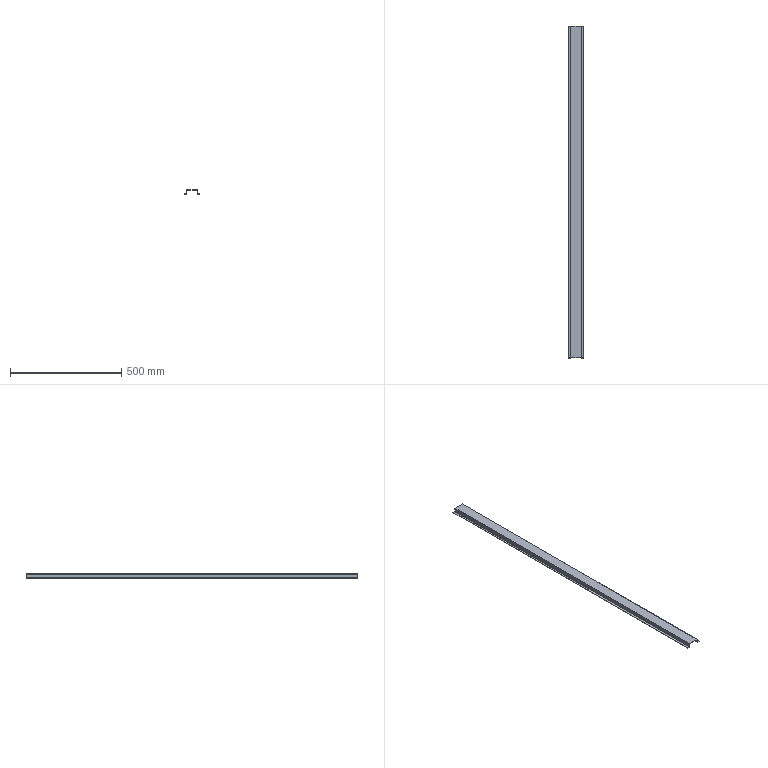Component | SolidWorks | AirFurnaceElectricalCabinet-RearSealingPlateAssembly-1_DoorPanelReinforcementPlate-L1490-1 | 1 solid | 38 faces | box 71.6 x 1490 x 18 mm | volume 183954 mm3 | plane 30 | cylinder 8 | commonest cylinder face diameters 3.9 x4 1.5 x4
STEP:
#1=COLOUR_RGB('',0.7922,0.8196,0.9333);
#2=FILL_AREA_STYLE_COLOUR('',#1);
#3=FILL_AREA_STYLE('',(#2));
#4=SURFACE_STYLE_FILL_AREA(#3);
#5=SURFACE_SIDE_STYLE('',(#4));
#6=SURFACE_STYLE_USAGE(.BOTH.,#5);
#7=PRESENTATION_STYLE_ASSIGNMENT((#6));
#8=CARTESIAN_POINT('',(0.9075,62.795,-9.272));
#9=VERTEX_POINT('',#8);
#10=CARTESIAN_POINT('',(-0.9075,62.795,-9.272));
#11=VERTEX_POINT('',#10);
#12=CARTESIAN_POINT('',(0.9843,62.795,-9.272));
#13=DIRECTION('',(-1.,0.,0.));
#14=VECTOR('',#13,39.37);
#15=LINE('',#12,#14);
#16=EDGE_CURVE('',#9,#11,#15,.T.);
#17=ORIENTED_EDGE('',*,*,#16,.F.);
#18=CARTESIAN_POINT('',(0.9075,62.795,-9.319));
#19=VERTEX_POINT('',#18);
#20=CARTESIAN_POINT('',(0.9075,62.795,-9.272));
#21=DIRECTION('',(0.,-0.,-1.));
#22=VECTOR('',#21,39.37);
#23=LINE('',#20,#22);
#24=EDGE_CURVE('',#9,#19,#23,.T.);
#25=ORIENTED_EDGE('',*,*,#24,.T.);
#26=CARTESIAN_POINT('',(-0.9075,62.795,-9.319));
#27=VERTEX_POINT('',#26);
#28=CARTESIAN_POINT('',(0.9843,62.795,-9.319));
#29=DIRECTION('',(-1.,0.,0.));
#30=VECTOR('',#29,39.37);
#31=LINE('',#28,#30);
#32=EDGE_CURVE('',#19,#27,#31,.T.);
#33=ORIENTED_EDGE('',*,*,#32,.T.);
#34=CARTESIAN_POINT('',(-0.9075,62.795,-9.319));
#35=DIRECTION('',(0.,0.,1.));
#36=VECTOR('',#35,39.37);
#37=LINE('',#34,#36);
#38=EDGE_CURVE('',#27,#11,#37,.T.);
#39=ORIENTED_EDGE('',*,*,#38,.T.);
#40=EDGE_LOOP('',(#17,#25,#33,#39));
#41=FACE_OUTER_BOUND('',#40,.T.);
#42=CARTESIAN_POINT('',(0.937,62.795,-9.348));
#43=DIRECTION('',(0.,1.,-0.));
#44=DIRECTION('',(-1.,0.,0.));
#45=AXIS2_PLACEMENT_3D('',#42,#43,#44);
#46=PLANE('',#45);
#47=ADVANCED_FACE('',(#41),#46,.T.);
#48=CARTESIAN_POINT('',(0.9075,4.134,-9.272));
#49=VERTEX_POINT('',#48);
#50=CARTESIAN_POINT('',(-0.9075,4.134,-9.272));
#51=VERTEX_POINT('',#50);
#52=CARTESIAN_POINT('',(0.9843,4.134,-9.272));
#53=DIRECTION('',(-1.,0.,0.));
#54=VECTOR('',#53,39.37);
#55=LINE('',#52,#54);
#56=EDGE_CURVE('',#49,#51,#55,.T.);
#57=ORIENTED_EDGE('',*,*,#56,.T.);
#58=CARTESIAN_POINT('',(-0.9075,4.134,-9.319));
#59=VERTEX_POINT('',#58);
#60=CARTESIAN_POINT('',(-0.9075,4.134,-9.272));
#61=DIRECTION('',(0.,-0.,-1.));
#62=VECTOR('',#61,39.37);
#63=LINE('',#60,#62);
#64=EDGE_CURVE('',#51,#59,#63,.T.);
#65=ORIENTED_EDGE('',*,*,#64,.T.);
#66=CARTESIAN_POINT('',(0.9075,4.134,-9.319));
#67=VERTEX_POINT('',#66);
#68=CARTESIAN_POINT('',(0.9843,4.134,-9.319));
#69=DIRECTION('',(-1.,0.,0.));
#70=VECTOR('',#69,39.37);
#71=LINE('',#68,#70);
#72=EDGE_CURVE('',#67,#59,#71,.T.);
#73=ORIENTED_EDGE('',*,*,#72,.F.);
#74=CARTESIAN_POINT('',(0.9075,4.134,-9.319));
#75=DIRECTION('',(0.,0.,1.));
#76=VECTOR('',#75,39.37);
#77=LINE('',#74,#76);
#78=EDGE_CURVE('',#67,#49,#77,.T.);
#79=ORIENTED_EDGE('',*,*,#78,.T.);
#80=EDGE_LOOP('',(#57,#65,#73,#79));
#81=FACE_OUTER_BOUND('',#80,.T.);
#82=CARTESIAN_POINT('',(-0.937,4.134,-9.348));
#83=DIRECTION('',(0.,-1.,0.));
#84=DIRECTION('',(1.,0.,0.));
#85=AXIS2_PLACEMENT_3D('',#82,#83,#84);
#86=PLANE('',#85);
#87=ADVANCED_FACE('',(#81),#86,.T.);
#88=ORIENTED_EDGE('',*,*,#56,.F.);
#89=CARTESIAN_POINT('',(0.9075,62.795,-9.272));
#90=DIRECTION('',(0.,-1.,0.));
#91=VECTOR('',#90,39.37);
#92=LINE('',#89,#91);
#93=EDGE_CURVE('',#9,#49,#92,.T.);
#94=ORIENTED_EDGE('',*,*,#93,.F.);
#95=ORIENTED_EDGE('',*,*,#16,.T.);
#96=CARTESIAN_POINT('',(-0.9075,62.795,-9.272));
#97=DIRECTION('',(0.,-1.,0.));
#98=VECTOR('',#97,39.37);
#99=LINE('',#96,#98);
#100=EDGE_CURVE('',#11,#51,#99,.T.);
#101=ORIENTED_EDGE('',*,*,#100,.T.);
#102=EDGE_LOOP('',(#88,#94,#95,#101));
#103=FACE_OUTER_BOUND('',#102,.T.);
#104=CARTESIAN_POINT('',(0.9843,62.795,-9.272));
#105=DIRECTION('',(0.,0.,1.));
#106=DIRECTION('',(1.,0.,0.));
#107=AXIS2_PLACEMENT_3D('',#104,#105,#106);
#108=PLANE('',#107);
#109=ADVANCED_FACE('',(#103),#108,.T.);
#110=ORIENTED_EDGE('',*,*,#72,.T.);
#111=CARTESIAN_POINT('',(-0.9075,62.795,-9.319));
#112=DIRECTION('',(0.,-1.,0.));
#113=VECTOR('',#112,39.37);
#114=LINE('',#111,#113);
#115=EDGE_CURVE('',#27,#59,#114,.T.);
#116=ORIENTED_EDGE('',*,*,#115,.F.);
#117=ORIENTED_EDGE('',*,*,#32,.F.);
#118=CARTESIAN_POINT('',(0.9075,62.795,-9.319));
#119=DIRECTION('',(0.,-1.,0.));
#120=VECTOR('',#119,39.37);
#121=LINE('',#118,#120);
#122=EDGE_CURVE('',#19,#67,#121,.T.);
#123=ORIENTED_EDGE('',*,*,#122,.T.);
#124=EDGE_LOOP('',(#110,#116,#117,#123));
#125=FACE_OUTER_BOUND('',#124,.T.);
#126=CARTESIAN_POINT('',(0.9843,62.795,-9.319));
#127=DIRECTION('',(0.,0.,1.));
#128=DIRECTION('',(1.,0.,0.));
#129=AXIS2_PLACEMENT_3D('',#126,#127,#128);
#130=PLANE('',#129);
#131=ADVANCED_FACE('',(#125),#130,.F.);
#132=ORIENTED_EDGE('',*,*,#38,.F.);
#133=CARTESIAN_POINT('',(-0.937,62.795,-9.348));
#134=VERTEX_POINT('',#133);
#135=CARTESIAN_POINT('',(-0.9075,62.795,-9.348));
#136=DIRECTION('',(0.,-1.,0.));
#137=DIRECTION('',(1.,0.,0.));
#138=AXIS2_PLACEMENT_3D('',#135,#136,#137);
#139=CIRCLE('',#138,0.02953);
#140=EDGE_CURVE('',#27,#134,#139,.T.);
#141=ORIENTED_EDGE('',*,*,#140,.T.);
#142=CARTESIAN_POINT('',(-0.9843,62.795,-9.348));
#143=VERTEX_POINT('',#142);
#144=CARTESIAN_POINT('',(-0.9843,62.795,-9.348));
#145=DIRECTION('',(1.,0.,0.));
#146=VECTOR('',#145,39.37);
#147=LINE('',#144,#146);
#148=EDGE_CURVE('',#143,#134,#147,.T.);
#149=ORIENTED_EDGE('',*,*,#148,.F.);
#150=CARTESIAN_POINT('',(-0.9075,62.795,-9.348));
#151=DIRECTION('',(0.,-1.,0.));
#152=DIRECTION('',(1.,0.,0.));
#153=AXIS2_PLACEMENT_3D('',#150,#151,#152);
#154=CIRCLE('',#153,0.07677);
#155=EDGE_CURVE('',#11,#143,#154,.T.);
#156=ORIENTED_EDGE('',*,*,#155,.F.);
#157=EDGE_LOOP('',(#132,#141,#149,#156));
#158=FACE_OUTER_BOUND('',#157,.T.);
#159=CARTESIAN_POINT('',(-0.9075,62.795,-9.348));
#160=DIRECTION('',(0.,1.,-0.));
#161=DIRECTION('',(-1.,0.,0.));
#162=AXIS2_PLACEMENT_3D('',#159,#160,#161);
#163=PLANE('',#162);
#164=ADVANCED_FACE('',(#158),#163,.T.);
#165=CARTESIAN_POINT('',(-0.937,4.134,-9.348));
#166=VERTEX_POINT('',#165);
#167=CARTESIAN_POINT('',(-0.9843,4.134,-9.348));
#168=VERTEX_POINT('',#167);
#169=CARTESIAN_POINT('',(-0.937,4.134,-9.348));
#170=DIRECTION('',(-1.,0.,0.));
#171=VECTOR('',#170,39.37);
#172=LINE('',#169,#171);
#173=EDGE_CURVE('',#166,#168,#172,.T.);
#174=ORIENTED_EDGE('',*,*,#173,.F.);
#175=CARTESIAN_POINT('',(-0.9075,4.134,-9.348));
#176=DIRECTION('',(0.,1.,-0.));
#177=DIRECTION('',(1.,0.,0.));
#178=AXIS2_PLACEMENT_3D('',#175,#176,#177);
#179=CIRCLE('',#178,0.02953);
#180=EDGE_CURVE('',#166,#59,#179,.T.);
#181=ORIENTED_EDGE('',*,*,#180,.T.);
#182=ORIENTED_EDGE('',*,*,#64,.F.);
#183=CARTESIAN_POINT('',(-0.9075,4.134,-9.348));
#184=DIRECTION('',(0.,1.,-0.));
#185=DIRECTION('',(-1.,0.,0.));
#186=AXIS2_PLACEMENT_3D('',#183,#184,#185);
#187=CIRCLE('',#186,0.07677);
#188=EDGE_CURVE('',#168,#51,#187,.T.);
#189=ORIENTED_EDGE('',*,*,#188,.F.);
#190=EDGE_LOOP('',(#174,#181,#182,#189));
#191=FACE_OUTER_BOUND('',#190,.T.);
#192=CARTESIAN_POINT('',(-0.9075,4.134,-9.348));
#193=DIRECTION('',(0.,-1.,0.));
#194=DIRECTION('',(1.,0.,0.));
#195=AXIS2_PLACEMENT_3D('',#192,#193,#194);
#196=PLANE('',#195);
#197=ADVANCED_FACE('',(#191),#196,.T.);
#198=ORIENTED_EDGE('',*,*,#188,.T.);
#199=ORIENTED_EDGE('',*,*,#100,.F.);
#200=ORIENTED_EDGE('',*,*,#155,.T.);
#201=CARTESIAN_POINT('',(-0.9843,62.795,-9.348));
#202=DIRECTION('',(0.,-1.,0.));
#203=VECTOR('',#202,39.37);
#204=LINE('',#201,#203);
#205=EDGE_CURVE('',#143,#168,#204,.T.);
#206=ORIENTED_EDGE('',*,*,#205,.T.);
#207=EDGE_LOOP('',(#198,#199,#200,#206));
#208=FACE_OUTER_BOUND('',#207,.T.);
#209=CARTESIAN_POINT('',(-0.9075,92.126,-9.348));
#210=DIRECTION('',(0.,-1.,0.));
#211=DIRECTION('',(1.,0.,0.));
#212=AXIS2_PLACEMENT_3D('',#209,#210,#211);
#213=CYLINDRICAL_SURFACE('',#212,0.07677);
#214=ADVANCED_FACE('',(#208),#213,.T.);
#215=ORIENTED_EDGE('',*,*,#180,.F.);
#216=CARTESIAN_POINT('',(-0.937,62.795,-9.348));
#217=DIRECTION('',(0.,-1.,0.));
#218=VECTOR('',#217,39.37);
#219=LINE('',#216,#218);
#220=EDGE_CURVE('',#134,#166,#219,.T.);
#221=ORIENTED_EDGE('',*,*,#220,.F.);
#222=ORIENTED_EDGE('',*,*,#140,.F.);
#223=ORIENTED_EDGE('',*,*,#115,.T.);
#224=EDGE_LOOP('',(#215,#221,#222,#223));
#225=FACE_OUTER_BOUND('',#224,.T.);
#226=CARTESIAN_POINT('',(-0.9075,92.126,-9.348));
#227=DIRECTION('',(0.,-1.,0.));
#228=DIRECTION('',(1.,0.,0.));
#229=AXIS2_PLACEMENT_3D('',#226,#227,#228);
#230=CYLINDRICAL_SURFACE('',#229,0.02953);
#231=ADVANCED_FACE('',(#225),#230,.F.);
#232=CARTESIAN_POINT('',(-1.409,4.134,-9.933));
#233=VERTEX_POINT('',#232);
#234=CARTESIAN_POINT('',(-1.409,4.134,-9.98));
#235=VERTEX_POINT('',#234);
#236=CARTESIAN_POINT('',(-1.409,4.134,-9.933));
#237=DIRECTION('',(0.,-0.,-1.));
#238=VECTOR('',#237,39.37);
#239=LINE('',#236,#238);
#240=EDGE_CURVE('',#233,#235,#239,.T.);
#241=ORIENTED_EDGE('',*,*,#240,.F.);
#242=CARTESIAN_POINT('',(-1.409,62.795,-9.933));
#243=VERTEX_POINT('',#242);
#244=CARTESIAN_POINT('',(-1.409,62.795,-9.933));
#245=DIRECTION('',(0.,-1.,0.));
#246=VECTOR('',#245,39.37);
#247=LINE('',#244,#246);
#248=EDGE_CURVE('',#243,#233,#247,.T.);
#249=ORIENTED_EDGE('',*,*,#248,.F.);
#250=CARTESIAN_POINT('',(-1.409,62.795,-9.98));
#251=VERTEX_POINT('',#250);
#252=CARTESIAN_POINT('',(-1.409,62.795,-9.933));
#253=DIRECTION('',(0.,-0.,-1.));
#254=VECTOR('',#253,39.37);
#255=LINE('',#252,#254);
#256=EDGE_CURVE('',#243,#251,#255,.T.);
#257=ORIENTED_EDGE('',*,*,#256,.T.);
#258=CARTESIAN_POINT('',(-1.409,62.795,-9.98));
#259=DIRECTION('',(0.,-1.,0.));
#260=VECTOR('',#259,39.37);
#261=LINE('',#258,#260);
#262=EDGE_CURVE('',#251,#235,#261,.T.);
#263=ORIENTED_EDGE('',*,*,#262,.T.);
#264=EDGE_LOOP('',(#241,#249,#257,#263));
#265=FACE_OUTER_BOUND('',#264,.T.);
#266=CARTESIAN_POINT('',(-1.409,62.795,-9.933));
#267=DIRECTION('',(-1.,0.,0.));
#268=DIRECTION('',(0.,-1.,0.));
#269=AXIS2_PLACEMENT_3D('',#266,#267,#268);
#270=PLANE('',#269);
#271=ADVANCED_FACE('',(#265),#270,.T.);
#272=CARTESIAN_POINT('',(-1.014,4.134,-9.98));
#273=VERTEX_POINT('',#272);
#274=CARTESIAN_POINT('',(-0.9843,4.134,-9.98));
#275=DIRECTION('',(-1.,0.,0.));
#276=VECTOR('',#275,39.37);
#277=LINE('',#274,#276);
#278=EDGE_CURVE('',#273,#235,#277,.T.);
#279=ORIENTED_EDGE('',*,*,#278,.F.);
#280=CARTESIAN_POINT('',(-1.014,4.134,-9.933));
#281=VERTEX_POINT('',#280);
#282=CARTESIAN_POINT('',(-1.014,4.134,-9.98));
#283=DIRECTION('',(0.,0.,1.));
#284=VECTOR('',#283,39.37);
#285=LINE('',#282,#284);
#286=EDGE_CURVE('',#273,#281,#285,.T.);
#287=ORIENTED_EDGE('',*,*,#286,.T.);
#288=CARTESIAN_POINT('',(-0.9843,4.134,-9.933));
#289=DIRECTION('',(-1.,0.,0.));
#290=VECTOR('',#289,39.37);
#291=LINE('',#288,#290);
#292=EDGE_CURVE('',#281,#233,#291,.T.);
#293=ORIENTED_EDGE('',*,*,#292,.T.);
#294=ORIENTED_EDGE('',*,*,#240,.T.);
#295=EDGE_LOOP('',(#279,#287,#293,#294));
#296=FACE_OUTER_BOUND('',#295,.T.);
#297=CARTESIAN_POINT('',(-1.014,4.134,-9.904));
#298=DIRECTION('',(0.,-1.,0.));
#299=DIRECTION('',(1.,0.,0.));
#300=AXIS2_PLACEMENT_3D('',#297,#298,#299);
#301=PLANE('',#300);
#302=ADVANCED_FACE('',(#296),#301,.T.);
#303=ORIENTED_EDGE('',*,*,#278,.T.);
#304=ORIENTED_EDGE('',*,*,#262,.F.);
#305=CARTESIAN_POINT('',(-1.014,62.795,-9.98));
#306=VERTEX_POINT('',#305);
#307=CARTESIAN_POINT('',(-0.9843,62.795,-9.98));
#308=DIRECTION('',(-1.,0.,0.));
#309=VECTOR('',#308,39.37);
#310=LINE('',#307,#309);
#311=EDGE_CURVE('',#306,#251,#310,.T.);
#312=ORIENTED_EDGE('',*,*,#311,.F.);
#313=CARTESIAN_POINT('',(-1.014,62.795,-9.98));
#314=DIRECTION('',(0.,-1.,0.));
#315=VECTOR('',#314,39.37);
#316=LINE('',#313,#315);
#317=EDGE_CURVE('',#306,#273,#316,.T.);
#318=ORIENTED_EDGE('',*,*,#317,.T.);
#319=EDGE_LOOP('',(#303,#304,#312,#318));
#320=FACE_OUTER_BOUND('',#319,.T.);
#321=CARTESIAN_POINT('',(-0.9843,62.795,-9.98));
#322=DIRECTION('',(0.,0.,1.));
#323=DIRECTION('',(1.,-0.,-0.));
#324=AXIS2_PLACEMENT_3D('',#321,#322,#323);
#325=PLANE('',#324);
#326=ADVANCED_FACE('',(#320),#325,.F.);
#327=CARTESIAN_POINT('',(-1.014,62.795,-9.933));
#328=VERTEX_POINT('',#327);
#329=CARTESIAN_POINT('',(-0.9843,62.795,-9.933));
#330=DIRECTION('',(-1.,0.,0.));
#331=VECTOR('',#330,39.37);
#332=LINE('',#329,#331);
#333=EDGE_CURVE('',#328,#243,#332,.T.);
#334=ORIENTED_EDGE('',*,*,#333,.F.);
#335=CARTESIAN_POINT('',(-1.014,62.795,-9.933));
#336=DIRECTION('',(0.,-0.,-1.));
#337=VECTOR('',#336,39.37);
#338=LINE('',#335,#337);
#339=EDGE_CURVE('',#328,#306,#338,.T.);
#340=ORIENTED_EDGE('',*,*,#339,.T.);
#341=ORIENTED_EDGE('',*,*,#311,.T.);
#342=ORIENTED_EDGE('',*,*,#256,.F.);
#343=EDGE_LOOP('',(#334,#340,#341,#342));
#344=FACE_OUTER_BOUND('',#343,.T.);
#345=CARTESIAN_POINT('',(-0.937,62.795,-9.904));
#346=DIRECTION('',(0.,1.,-0.));
#347=DIRECTION('',(-1.,0.,0.));
#348=AXIS2_PLACEMENT_3D('',#345,#346,#347);
#349=PLANE('',#348);
#350=ADVANCED_FACE('',(#344),#349,.T.);
#351=ORIENTED_EDGE('',*,*,#292,.F.);
#352=CARTESIAN_POINT('',(-1.014,62.795,-9.933));
#353=DIRECTION('',(0.,-1.,0.));
#354=VECTOR('',#353,39.37);
#355=LINE('',#352,#354);
#356=EDGE_CURVE('',#328,#281,#355,.T.);
#357=ORIENTED_EDGE('',*,*,#356,.F.);
#358=ORIENTED_EDGE('',*,*,#333,.T.);
#359=ORIENTED_EDGE('',*,*,#248,.T.);
#360=EDGE_LOOP('',(#351,#357,#358,#359));
#361=FACE_OUTER_BOUND('',#360,.T.);
#362=CARTESIAN_POINT('',(-0.9843,62.795,-9.933));
#363=DIRECTION('',(0.,0.,1.));
#364=DIRECTION('',(1.,-0.,-0.));
#365=AXIS2_PLACEMENT_3D('',#362,#363,#364);
#366=PLANE('',#365);
#367=ADVANCED_FACE('',(#361),#366,.T.);
#368=ORIENTED_EDGE('',*,*,#286,.F.);
#369=CARTESIAN_POINT('',(-0.937,4.134,-9.904));
#370=VERTEX_POINT('',#369);
#371=CARTESIAN_POINT('',(-1.014,4.134,-9.904));
#372=DIRECTION('',(0.,-1.,0.));
#373=DIRECTION('',(0.,0.,1.));
#374=AXIS2_PLACEMENT_3D('',#371,#372,#373);
#375=CIRCLE('',#374,0.07677);
#376=EDGE_CURVE('',#273,#370,#375,.T.);
#377=ORIENTED_EDGE('',*,*,#376,.T.);
#378=CARTESIAN_POINT('',(-0.9843,4.134,-9.904));
#379=VERTEX_POINT('',#378);
#380=CARTESIAN_POINT('',(-0.9843,4.134,-9.904));
#381=DIRECTION('',(1.,0.,0.));
#382=VECTOR('',#381,39.37);
#383=LINE('',#380,#382);
#384=EDGE_CURVE('',#379,#370,#383,.T.);
#385=ORIENTED_EDGE('',*,*,#384,.F.);
#386=CARTESIAN_POINT('',(-1.014,4.134,-9.904));
#387=DIRECTION('',(0.,-1.,0.));
#388=DIRECTION('',(0.,0.,1.));
#389=AXIS2_PLACEMENT_3D('',#386,#387,#388);
#390=CIRCLE('',#389,0.02953);
#391=EDGE_CURVE('',#281,#379,#390,.T.);
#392=ORIENTED_EDGE('',*,*,#391,.F.);
#393=EDGE_LOOP('',(#368,#377,#385,#392));
#394=FACE_OUTER_BOUND('',#393,.T.);
#395=CARTESIAN_POINT('',(-1.014,4.134,-9.904));
#396=DIRECTION('',(0.,1.,-0.));
#397=DIRECTION('',(-0.,-0.,-1.));
#398=AXIS2_PLACEMENT_3D('',#395,#396,#397);
#399=PLANE('',#398);
#400=ADVANCED_FACE('',(#394),#399,.F.);
#401=ORIENTED_EDGE('',*,*,#376,.F.);
#402=ORIENTED_EDGE('',*,*,#317,.F.);
#403=CARTESIAN_POINT('',(-0.937,62.795,-9.904));
#404=VERTEX_POINT('',#403);
#405=CARTESIAN_POINT('',(-1.014,62.795,-9.904));
#406=DIRECTION('',(0.,1.,-0.));
#407=DIRECTION('',(0.,0.,1.));
#408=AXIS2_PLACEMENT_3D('',#405,#406,#407);
#409=CIRCLE('',#408,0.07677);
#410=EDGE_CURVE('',#404,#306,#409,.T.);
#411=ORIENTED_EDGE('',*,*,#410,.F.);
#412=CARTESIAN_POINT('',(-0.937,62.795,-9.904));
#413=DIRECTION('',(0.,-1.,0.));
#414=VECTOR('',#413,39.37);
#415=LINE('',#412,#414);
#416=EDGE_CURVE('',#404,#370,#415,.T.);
#417=ORIENTED_EDGE('',*,*,#416,.T.);
#418=EDGE_LOOP('',(#401,#402,#411,#417));
#419=FACE_OUTER_BOUND('',#418,.T.);
#420=CARTESIAN_POINT('',(-1.014,92.126,-9.904));
#421=DIRECTION('',(0.,-1.,0.));
#422=DIRECTION('',(0.,0.,1.));
#423=AXIS2_PLACEMENT_3D('',#420,#421,#422);
#424=CYLINDRICAL_SURFACE('',#423,0.07677);
#425=ADVANCED_FACE('',(#419),#424,.T.);
#426=CARTESIAN_POINT('',(-0.9843,62.795,-9.904));
#427=VERTEX_POINT('',#426);
#428=CARTESIAN_POINT('',(-0.937,62.795,-9.904));
#429=DIRECTION('',(-1.,-0.,-0.));
#430=VECTOR('',#429,39.37);
#431=LINE('',#428,#430);
#432=EDGE_CURVE('',#404,#427,#431,.T.);
#433=ORIENTED_EDGE('',*,*,#432,.F.);
#434=ORIENTED_EDGE('',*,*,#410,.T.);
#435=ORIENTED_EDGE('',*,*,#339,.F.);
#436=CARTESIAN_POINT('',(-1.014,62.795,-9.904));
#437=DIRECTION('',(0.,1.,-0.));
#438=DIRECTION('',(0.,0.,-1.));
#439=AXIS2_PLACEMENT_3D('',#436,#437,#438);
#440=CIRCLE('',#439,0.02953);
#441=EDGE_CURVE('',#427,#328,#440,.T.);
#442=ORIENTED_EDGE('',*,*,#441,.F.);
#443=EDGE_LOOP('',(#433,#434,#435,#442));
#444=FACE_OUTER_BOUND('',#443,.T.);
#445=CARTESIAN_POINT('',(-1.014,62.795,-9.904));
#446=DIRECTION('',(0.,-1.,0.));
#447=DIRECTION('',(0.,0.,1.));
#448=AXIS2_PLACEMENT_3D('',#445,#446,#447);
#449=PLANE('',#448);
#450=ADVANCED_FACE('',(#444),#449,.F.);
#451=ORIENTED_EDGE('',*,*,#391,.T.);
#452=CARTESIAN_POINT('',(-0.9843,62.795,-9.904));
#453=DIRECTION('',(0.,-1.,0.));
#454=VECTOR('',#453,39.37);
#455=LINE('',#452,#454);
#456=EDGE_CURVE('',#427,#379,#455,.T.);
#457=ORIENTED_EDGE('',*,*,#456,.F.);
#458=ORIENTED_EDGE('',*,*,#441,.T.);
#459=ORIENTED_EDGE('',*,*,#356,.T.);
#460=EDGE_LOOP('',(#451,#457,#458,#459));
#461=FACE_OUTER_BOUND('',#460,.T.);
#462=CARTESIAN_POINT('',(-1.014,92.126,-9.904));
#463=DIRECTION('',(0.,-1.,0.));
#464=DIRECTION('',(0.,0.,1.));
#465=AXIS2_PLACEMENT_3D('',#462,#463,#464);
#466=CYLINDRICAL_SURFACE('',#465,0.02953);
#467=ADVANCED_FACE('',(#461),#466,.F.);
#468=CARTESIAN_POINT('',(-0.9843,4.134,-9.272));
#469=DIRECTION('',(0.,-0.,-1.));
#470=VECTOR('',#469,39.37);
#471=LINE('',#468,#470);
#472=EDGE_CURVE('',#168,#379,#471,.T.);
#473=ORIENTED_EDGE('',*,*,#472,.F.);
#474=ORIENTED_EDGE('',*,*,#205,.F.);
#475=CARTESIAN_POINT('',(-0.9843,62.795,-9.272));
#476=DIRECTION('',(0.,-0.,-1.));
#477=VECTOR('',#476,39.37);
#478=LINE('',#475,#477);
#479=EDGE_CURVE('',#143,#427,#478,.T.);
#480=ORIENTED_EDGE('',*,*,#479,.T.);
#481=ORIENTED_EDGE('',*,*,#456,.T.);
#482=EDGE_LOOP('',(#473,#474,#480,#481));
#483=FACE_OUTER_BOUND('',#482,.T.);
#484=CARTESIAN_POINT('',(-0.9843,62.795,-9.272));
#485=DIRECTION('',(-1.,0.,0.));
#486=DIRECTION('',(0.,-1.,0.));
#487=AXIS2_PLACEMENT_3D('',#484,#485,#486);
#488=PLANE('',#487);
#489=ADVANCED_FACE('',(#483),#488,.T.);
#490=ORIENTED_EDGE('',*,*,#479,.F.);
#491=ORIENTED_EDGE('',*,*,#148,.T.);
#492=CARTESIAN_POINT('',(-0.937,62.795,-9.272));
#493=DIRECTION('',(0.,-0.,-1.));
#494=VECTOR('',#493,39.37);
#495=LINE('',#492,#494);
#496=EDGE_CURVE('',#134,#404,#495,.T.);
#497=ORIENTED_EDGE('',*,*,#496,.T.);
#498=ORIENTED_EDGE('',*,*,#432,.T.);
#499=EDGE_LOOP('',(#490,#491,#497,#498));
#500=FACE_OUTER_BOUND('',#499,.T.);
#501=CARTESIAN_POINT('',(-0.9075,62.795,-9.319));
#502=DIRECTION('',(0.,1.,-0.));
#503=DIRECTION('',(-1.,0.,0.));
#504=AXIS2_PLACEMENT_3D('',#501,#502,#503);
#505=PLANE('',#504);
#506=ADVANCED_FACE('',(#500),#505,.T.);
#507=CARTESIAN_POINT('',(-0.937,4.134,-9.272));
#508=DIRECTION('',(0.,-0.,-1.));
#509=VECTOR('',#508,39.37);
#510=LINE('',#507,#509);
#511=EDGE_CURVE('',#166,#370,#510,.T.);
#512=ORIENTED_EDGE('',*,*,#511,.T.);
#513=ORIENTED_EDGE('',*,*,#416,.F.);
#514=ORIENTED_EDGE('',*,*,#496,.F.);
#515=ORIENTED_EDGE('',*,*,#220,.T.);
#516=EDGE_LOOP('',(#512,#513,#514,#515));
#517=FACE_OUTER_BOUND('',#516,.T.);
#518=CARTESIAN_POINT('',(-0.937,62.795,-9.272));
#519=DIRECTION('',(-1.,0.,0.));
#520=DIRECTION('',(0.,-1.,0.));
#521=AXIS2_PLACEMENT_3D('',#518,#519,#520);
#522=PLANE('',#521);
#523=ADVANCED_FACE('',(#517),#522,.F.);
#524=ORIENTED_EDGE('',*,*,#472,.T.);
#525=ORIENTED_EDGE('',*,*,#384,.T.);
#526=ORIENTED_EDGE('',*,*,#511,.F.);
#527=ORIENTED_EDGE('',*,*,#173,.T.);
#528=EDGE_LOOP('',(#524,#525,#526,#527));
#529=FACE_OUTER_BOUND('',#528,.T.);
#530=CARTESIAN_POINT('',(-1.014,4.134,-9.98));
#531=DIRECTION('',(0.,-1.,0.));
#532=DIRECTION('',(1.,0.,0.));
#533=AXIS2_PLACEMENT_3D('',#530,#531,#532);
#534=PLANE('',#533);
#535=ADVANCED_FACE('',(#529),#534,.T.);
#536=CARTESIAN_POINT('',(0.937,62.795,-9.348));
#537=VERTEX_POINT('',#536);
#538=CARTESIAN_POINT('',(0.9843,62.795,-9.348));
#539=VERTEX_POINT('',#538);
#540=CARTESIAN_POINT('',(0.937,62.795,-9.348));
#541=DIRECTION('',(1.,0.,0.));
#542=VECTOR('',#541,39.37);
#543=LINE('',#540,#542);
#544=EDGE_CURVE('',#537,#539,#543,.T.);
#545=ORIENTED_EDGE('',*,*,#544,.F.);
#546=CARTESIAN_POINT('',(0.9075,62.795,-9.348));
#547=DIRECTION('',(0.,-1.,0.));
#548=DIRECTION('',(-1.,0.,0.));
#549=AXIS2_PLACEMENT_3D('',#546,#547,#548);
#550=CIRCLE('',#549,0.02953);
#551=EDGE_CURVE('',#537,#19,#550,.T.);
#552=ORIENTED_EDGE('',*,*,#551,.T.);
#553=ORIENTED_EDGE('',*,*,#24,.F.);
#554=CARTESIAN_POINT('',(0.9075,62.795,-9.348));
#555=DIRECTION('',(0.,-1.,0.));
#556=DIRECTION('',(1.,0.,0.));
#557=AXIS2_PLACEMENT_3D('',#554,#555,#556);
#558=CIRCLE('',#557,0.07677);
#559=EDGE_CURVE('',#539,#9,#558,.T.);
#560=ORIENTED_EDGE('',*,*,#559,.F.);
#561=EDGE_LOOP('',(#545,#552,#553,#560));
#562=FACE_OUTER_BOUND('',#561,.T.);
#563=CARTESIAN_POINT('',(0.9075,62.795,-9.348));
#564=DIRECTION('',(0.,1.,-0.));
#565=DIRECTION('',(-1.,0.,0.));
#566=AXIS2_PLACEMENT_3D('',#563,#564,#565);
#567=PLANE('',#566);
#568=ADVANCED_FACE('',(#562),#567,.T.);
#569=ORIENTED_EDGE('',*,*,#78,.F.);
#570=CARTESIAN_POINT('',(0.937,4.134,-9.348));
#571=VERTEX_POINT('',#570);
#572=CARTESIAN_POINT('',(0.9075,4.134,-9.348));
#573=DIRECTION('',(0.,1.,-0.));
#574=DIRECTION('',(-1.,0.,0.));
#575=AXIS2_PLACEMENT_3D('',#572,#573,#574);
#576=CIRCLE('',#575,0.02953);
#577=EDGE_CURVE('',#67,#571,#576,.T.);
#578=ORIENTED_EDGE('',*,*,#577,.T.);
#579=CARTESIAN_POINT('',(0.9843,4.134,-9.348));
#580=VERTEX_POINT('',#579);
#581=CARTESIAN_POINT('',(0.9843,4.134,-9.348));
#582=DIRECTION('',(-1.,0.,0.));
#583=VECTOR('',#582,39.37);
#584=LINE('',#581,#583);
#585=EDGE_CURVE('',#580,#571,#584,.T.);
#586=ORIENTED_EDGE('',*,*,#585,.F.);
#587=CARTESIAN_POINT('',(0.9075,4.134,-9.348));
#588=DIRECTION('',(0.,1.,-0.));
#589=DIRECTION('',(-1.,0.,0.));
#590=AXIS2_PLACEMENT_3D('',#587,#588,#589);
#591=CIRCLE('',#590,0.07677);
#592=EDGE_CURVE('',#49,#580,#591,.T.);
#593=ORIENTED_EDGE('',*,*,#592,.F.);
#594=EDGE_LOOP('',(#569,#578,#586,#593));
#595=FACE_OUTER_BOUND('',#594,.T.);
#596=CARTESIAN_POINT('',(0.9075,4.134,-9.348));
#597=DIRECTION('',(0.,-1.,0.));
#598=DIRECTION('',(1.,0.,0.));
#599=AXIS2_PLACEMENT_3D('',#596,#597,#598);
#600=PLANE('',#599);
#601=ADVANCED_FACE('',(#595),#600,.T.);
#602=ORIENTED_EDGE('',*,*,#592,.T.);
#603=CARTESIAN_POINT('',(0.9843,62.795,-9.348));
#604=DIRECTION('',(0.,-1.,0.));
#605=VECTOR('',#604,39.37);
#606=LINE('',#603,#605);
#607=EDGE_CURVE('',#539,#580,#606,.T.);
#608=ORIENTED_EDGE('',*,*,#607,.F.);
#609=ORIENTED_EDGE('',*,*,#559,.T.);
#610=ORIENTED_EDGE('',*,*,#93,.T.);
#611=EDGE_LOOP('',(#602,#608,#609,#610));
#612=FACE_OUTER_BOUND('',#611,.T.);
#613=CARTESIAN_POINT('',(0.9075,-25.197,-9.348));
#614=DIRECTION('',(0.,1.,-0.));
#615=DIRECTION('',(-1.,0.,0.));
#616=AXIS2_PLACEMENT_3D('',#613,#614,#615);
#617=CYLINDRICAL_SURFACE('',#616,0.07677);
#618=ADVANCED_FACE('',(#612),#617,.T.);
#619=ORIENTED_EDGE('',*,*,#577,.F.);
#620=ORIENTED_EDGE('',*,*,#122,.F.);
#621=ORIENTED_EDGE('',*,*,#551,.F.);
#622=CARTESIAN_POINT('',(0.937,62.795,-9.348));
#623=DIRECTION('',(0.,-1.,0.));
#624=VECTOR('',#623,39.37);
#625=LINE('',#622,#624);
#626=EDGE_CURVE('',#537,#571,#625,.T.);
#627=ORIENTED_EDGE('',*,*,#626,.T.);
#628=EDGE_LOOP('',(#619,#620,#621,#627));
#629=FACE_OUTER_BOUND('',#628,.T.);
#630=CARTESIAN_POINT('',(0.9075,-25.197,-9.348));
#631=DIRECTION('',(0.,1.,-0.));
#632=DIRECTION('',(-1.,0.,0.));
#633=AXIS2_PLACEMENT_3D('',#630,#631,#632);
#634=CYLINDRICAL_SURFACE('',#633,0.02953);
#635=ADVANCED_FACE('',(#629),#634,.F.);
#636=CARTESIAN_POINT('',(0.9843,4.134,-9.904));
#637=VERTEX_POINT('',#636);
#638=CARTESIAN_POINT('',(0.9843,4.134,-9.933));
#639=DIRECTION('',(0.,0.,1.));
#640=VECTOR('',#639,39.37);
#641=LINE('',#638,#640);
#642=EDGE_CURVE('',#637,#580,#641,.T.);
#643=ORIENTED_EDGE('',*,*,#642,.F.);
#644=CARTESIAN_POINT('',(0.9843,62.795,-9.904));
#645=VERTEX_POINT('',#644);
#646=CARTESIAN_POINT('',(0.9843,62.795,-9.904));
#647=DIRECTION('',(0.,-1.,0.));
#648=VECTOR('',#647,39.37);
#649=LINE('',#646,#648);
#650=EDGE_CURVE('',#645,#637,#649,.T.);
#651=ORIENTED_EDGE('',*,*,#650,.F.);
#652=CARTESIAN_POINT('',(0.9843,62.795,-9.933));
#653=DIRECTION('',(0.,0.,1.));
#654=VECTOR('',#653,39.37);
#655=LINE('',#652,#654);
#656=EDGE_CURVE('',#645,#539,#655,.T.);
#657=ORIENTED_EDGE('',*,*,#656,.T.);
#658=ORIENTED_EDGE('',*,*,#607,.T.);
#659=EDGE_LOOP('',(#643,#651,#657,#658));
#660=FACE_OUTER_BOUND('',#659,.T.);
#661=CARTESIAN_POINT('',(0.9843,62.795,-9.933));
#662=DIRECTION('',(1.,0.,0.));
#663=DIRECTION('',(0.,1.,-0.));
#664=AXIS2_PLACEMENT_3D('',#661,#662,#663);
#665=PLANE('',#664);
#666=ADVANCED_FACE('',(#660),#665,.T.);
#667=ORIENTED_EDGE('',*,*,#642,.T.);
#668=ORIENTED_EDGE('',*,*,#585,.T.);
#669=CARTESIAN_POINT('',(0.937,4.134,-9.904));
#670=VERTEX_POINT('',#669);
#671=CARTESIAN_POINT('',(0.937,4.134,-9.933));
#672=DIRECTION('',(0.,0.,1.));
#673=VECTOR('',#672,39.37);
#674=LINE('',#671,#673);
#675=EDGE_CURVE('',#670,#571,#674,.T.);
#676=ORIENTED_EDGE('',*,*,#675,.F.);
#677=CARTESIAN_POINT('',(0.937,4.134,-9.904));
#678=DIRECTION('',(1.,0.,0.));
#679=VECTOR('',#678,39.37);
#680=LINE('',#677,#679);
#681=EDGE_CURVE('',#670,#637,#680,.T.);
#682=ORIENTED_EDGE('',*,*,#681,.T.);
#683=EDGE_LOOP('',(#667,#668,#676,#682));
#684=FACE_OUTER_BOUND('',#683,.T.);
#685=CARTESIAN_POINT('',(0.9075,4.134,-9.319));
#686=DIRECTION('',(0.,-1.,0.));
#687=DIRECTION('',(1.,0.,0.));
#688=AXIS2_PLACEMENT_3D('',#685,#686,#687);
#689=PLANE('',#688);
#690=ADVANCED_FACE('',(#684),#689,.T.);
#691=ORIENTED_EDGE('',*,*,#675,.T.);
#692=ORIENTED_EDGE('',*,*,#626,.F.);
#693=CARTESIAN_POINT('',(0.937,62.795,-9.904));
#694=VERTEX_POINT('',#693);
#695=CARTESIAN_POINT('',(0.937,62.795,-9.933));
#696=DIRECTION('',(0.,0.,1.));
#697=VECTOR('',#696,39.37);
#698=LINE('',#695,#697);
#699=EDGE_CURVE('',#694,#537,#698,.T.);
#700=ORIENTED_EDGE('',*,*,#699,.F.);
#701=CARTESIAN_POINT('',(0.937,62.795,-9.904));
#702=DIRECTION('',(0.,-1.,0.));
#703=VECTOR('',#702,39.37);
#704=LINE('',#701,#703);
#705=EDGE_CURVE('',#694,#670,#704,.T.);
#706=ORIENTED_EDGE('',*,*,#705,.T.);
#707=EDGE_LOOP('',(#691,#692,#700,#706));
#708=FACE_OUTER_BOUND('',#707,.T.);
#709=CARTESIAN_POINT('',(0.937,62.795,-9.933));
#710=DIRECTION('',(1.,0.,0.));
#711=DIRECTION('',(0.,1.,-0.));
#712=AXIS2_PLACEMENT_3D('',#709,#710,#711);
#713=PLANE('',#712);
#714=ADVANCED_FACE('',(#708),#713,.F.);
#715=ORIENTED_EDGE('',*,*,#656,.F.);
#716=CARTESIAN_POINT('',(0.9843,62.795,-9.904));
#717=DIRECTION('',(-1.,0.,0.));
#718=VECTOR('',#717,39.37);
#719=LINE('',#716,#718);
#720=EDGE_CURVE('',#645,#694,#719,.T.);
#721=ORIENTED_EDGE('',*,*,#720,.T.);
#722=ORIENTED_EDGE('',*,*,#699,.T.);
#723=ORIENTED_EDGE('',*,*,#544,.T.);
#724=EDGE_LOOP('',(#715,#721,#722,#723));
#725=FACE_OUTER_BOUND('',#724,.T.);
#726=CARTESIAN_POINT('',(1.014,62.795,-9.98));
#727=DIRECTION('',(0.,1.,-0.));
#728=DIRECTION('',(-1.,0.,0.));
#729=AXIS2_PLACEMENT_3D('',#726,#727,#728);
#730=PLANE('',#729);
#731=ADVANCED_FACE('',(#725),#730,.T.);
#732=CARTESIAN_POINT('',(1.014,62.795,-9.98));
#733=VERTEX_POINT('',#732);
#734=CARTESIAN_POINT('',(1.014,62.795,-9.933));
#735=VERTEX_POINT('',#734);
#736=CARTESIAN_POINT('',(1.014,62.795,-9.98));
#737=DIRECTION('',(0.,0.,1.));
#738=VECTOR('',#737,39.37);
#739=LINE('',#736,#738);
#740=EDGE_CURVE('',#733,#735,#739,.T.);
#741=ORIENTED_EDGE('',*,*,#740,.F.);
#742=CARTESIAN_POINT('',(1.014,62.795,-9.904));
#743=DIRECTION('',(0.,1.,-0.));
#744=DIRECTION('',(-1.,0.,0.));
#745=AXIS2_PLACEMENT_3D('',#742,#743,#744);
#746=CIRCLE('',#745,0.07677);
#747=EDGE_CURVE('',#733,#694,#746,.T.);
#748=ORIENTED_EDGE('',*,*,#747,.T.);
#749=ORIENTED_EDGE('',*,*,#720,.F.);
#750=CARTESIAN_POINT('',(1.014,62.795,-9.904));
#751=DIRECTION('',(0.,1.,-0.));
#752=DIRECTION('',(-1.,0.,0.));
#753=AXIS2_PLACEMENT_3D('',#750,#751,#752);
#754=CIRCLE('',#753,0.02953);
#755=EDGE_CURVE('',#735,#645,#754,.T.);
#756=ORIENTED_EDGE('',*,*,#755,.F.);
#757=EDGE_LOOP('',(#741,#748,#749,#756));
#758=FACE_OUTER_BOUND('',#757,.T.);
#759=CARTESIAN_POINT('',(1.014,62.795,-9.904));
#760=DIRECTION('',(0.,-1.,0.));
#761=DIRECTION('',(1.,0.,0.));
#762=AXIS2_PLACEMENT_3D('',#759,#760,#761);
#763=PLANE('',#762);
#764=ADVANCED_FACE('',(#758),#763,.F.);
#765=ORIENTED_EDGE('',*,*,#681,.F.);
#766=CARTESIAN_POINT('',(1.014,4.134,-9.98));
#767=VERTEX_POINT('',#766);
#768=CARTESIAN_POINT('',(1.014,4.134,-9.904));
#769=DIRECTION('',(0.,-1.,0.));
#770=DIRECTION('',(-1.,0.,0.));
#771=AXIS2_PLACEMENT_3D('',#768,#769,#770);
#772=CIRCLE('',#771,0.07677);
#773=EDGE_CURVE('',#670,#767,#772,.T.);
#774=ORIENTED_EDGE('',*,*,#773,.T.);
#775=CARTESIAN_POINT('',(1.014,4.134,-9.933));
#776=VERTEX_POINT('',#775);
#777=CARTESIAN_POINT('',(1.014,4.134,-9.933));
#778=DIRECTION('',(0.,-0.,-1.));
#779=VECTOR('',#778,39.37);
#780=LINE('',#777,#779);
#781=EDGE_CURVE('',#776,#767,#780,.T.);
#782=ORIENTED_EDGE('',*,*,#781,.F.);
#783=CARTESIAN_POINT('',(1.014,4.134,-9.904));
#784=DIRECTION('',(0.,-1.,0.));
#785=DIRECTION('',(1.,0.,0.));
#786=AXIS2_PLACEMENT_3D('',#783,#784,#785);
#787=CIRCLE('',#786,0.02953);
#788=EDGE_CURVE('',#637,#776,#787,.T.);
#789=ORIENTED_EDGE('',*,*,#788,.F.);
#790=EDGE_LOOP('',(#765,#774,#782,#789));
#791=FACE_OUTER_BOUND('',#790,.T.);
#792=CARTESIAN_POINT('',(1.014,4.134,-9.904));
#793=DIRECTION('',(0.,1.,-0.));
#794=DIRECTION('',(-1.,0.,0.));
#795=AXIS2_PLACEMENT_3D('',#792,#793,#794);
#796=PLANE('',#795);
#797=ADVANCED_FACE('',(#791),#796,.F.);
#798=ORIENTED_EDGE('',*,*,#788,.T.);
#799=CARTESIAN_POINT('',(1.014,62.795,-9.933));
#800=DIRECTION('',(0.,-1.,0.));
#801=VECTOR('',#800,39.37);
#802=LINE('',#799,#801);
#803=EDGE_CURVE('',#735,#776,#802,.T.);
#804=ORIENTED_EDGE('',*,*,#803,.F.);
#805=ORIENTED_EDGE('',*,*,#755,.T.);
#806=ORIENTED_EDGE('',*,*,#650,.T.);
#807=EDGE_LOOP('',(#798,#804,#805,#806));
#808=FACE_OUTER_BOUND('',#807,.T.);
#809=CARTESIAN_POINT('',(1.014,-25.197,-9.904));
#810=DIRECTION('',(0.,1.,-0.));
#811=DIRECTION('',(-1.,0.,0.));
#812=AXIS2_PLACEMENT_3D('',#809,#810,#811);
#813=CYLINDRICAL_SURFACE('',#812,0.02953);
#814=ADVANCED_FACE('',(#808),#813,.F.);
#815=ORIENTED_EDGE('',*,*,#773,.F.);
#816=ORIENTED_EDGE('',*,*,#705,.F.);
#817=ORIENTED_EDGE('',*,*,#747,.F.);
#818=CARTESIAN_POINT('',(1.014,62.795,-9.98));
#819=DIRECTION('',(0.,-1.,0.));
#820=VECTOR('',#819,39.37);
#821=LINE('',#818,#820);
#822=EDGE_CURVE('',#733,#767,#821,.T.);
#823=ORIENTED_EDGE('',*,*,#822,.T.);
#824=EDGE_LOOP('',(#815,#816,#817,#823));
#825=FACE_OUTER_BOUND('',#824,.T.);
#826=CARTESIAN_POINT('',(1.014,-25.197,-9.904));
#827=DIRECTION('',(0.,1.,-0.));
#828=DIRECTION('',(-1.,0.,0.));
#829=AXIS2_PLACEMENT_3D('',#826,#827,#828);
#830=CYLINDRICAL_SURFACE('',#829,0.07677);
#831=ADVANCED_FACE('',(#825),#830,.T.);
#832=CARTESIAN_POINT('',(1.409,4.134,-9.98));
#833=VERTEX_POINT('',#832);
#834=CARTESIAN_POINT('',(1.409,4.134,-9.933));
#835=VERTEX_POINT('',#834);
#836=CARTESIAN_POINT('',(1.409,4.134,-9.98));
#837=DIRECTION('',(0.,0.,1.));
#838=VECTOR('',#837,39.37);
#839=LINE('',#836,#838);
#840=EDGE_CURVE('',#833,#835,#839,.T.);
#841=ORIENTED_EDGE('',*,*,#840,.F.);
#842=CARTESIAN_POINT('',(1.409,62.795,-9.98));
#843=VERTEX_POINT('',#842);
#844=CARTESIAN_POINT('',(1.409,62.795,-9.98));
#845=DIRECTION('',(0.,-1.,0.));
#846=VECTOR('',#845,39.37);
#847=LINE('',#844,#846);
#848=EDGE_CURVE('',#843,#833,#847,.T.);
#849=ORIENTED_EDGE('',*,*,#848,.F.);
#850=CARTESIAN_POINT('',(1.409,62.795,-9.933));
#851=VERTEX_POINT('',#850);
#852=CARTESIAN_POINT('',(1.409,62.795,-9.98));
#853=DIRECTION('',(0.,0.,1.));
#854=VECTOR('',#853,39.37);
#855=LINE('',#852,#854);
#856=EDGE_CURVE('',#843,#851,#855,.T.);
#857=ORIENTED_EDGE('',*,*,#856,.T.);
#858=CARTESIAN_POINT('',(1.409,62.795,-9.933));
#859=DIRECTION('',(0.,-1.,0.));
#860=VECTOR('',#859,39.37);
#861=LINE('',#858,#860);
#862=EDGE_CURVE('',#851,#835,#861,.T.);
#863=ORIENTED_EDGE('',*,*,#862,.T.);
#864=EDGE_LOOP('',(#841,#849,#857,#863));
#865=FACE_OUTER_BOUND('',#864,.T.);
#866=CARTESIAN_POINT('',(1.409,62.795,-9.98));
#867=DIRECTION('',(1.,0.,0.));
#868=DIRECTION('',(0.,1.,-0.));
#869=AXIS2_PLACEMENT_3D('',#866,#867,#868);
#870=PLANE('',#869);
#871=ADVANCED_FACE('',(#865),#870,.T.);
#872=CARTESIAN_POINT('',(1.409,4.134,-9.933));
#873=DIRECTION('',(-1.,-0.,-0.));
#874=VECTOR('',#873,39.37);
#875=LINE('',#872,#874);
#876=EDGE_CURVE('',#835,#776,#875,.T.);
#877=ORIENTED_EDGE('',*,*,#876,.F.);
#878=ORIENTED_EDGE('',*,*,#862,.F.);
#879=CARTESIAN_POINT('',(1.409,62.795,-9.933));
#880=DIRECTION('',(-1.,-0.,-0.));
#881=VECTOR('',#880,39.37);
#882=LINE('',#879,#881);
#883=EDGE_CURVE('',#851,#735,#882,.T.);
#884=ORIENTED_EDGE('',*,*,#883,.T.);
#885=ORIENTED_EDGE('',*,*,#803,.T.);
#886=EDGE_LOOP('',(#877,#878,#884,#885));
#887=FACE_OUTER_BOUND('',#886,.T.);
#888=CARTESIAN_POINT('',(1.409,62.795,-9.933));
#889=DIRECTION('',(-0.,0.,1.));
#890=DIRECTION('',(1.,0.,0.));
#891=AXIS2_PLACEMENT_3D('',#888,#889,#890);
#892=PLANE('',#891);
#893=ADVANCED_FACE('',(#887),#892,.T.);
#894=ORIENTED_EDGE('',*,*,#876,.T.);
#895=ORIENTED_EDGE('',*,*,#781,.T.);
#896=CARTESIAN_POINT('',(1.409,4.134,-9.98));
#897=DIRECTION('',(-1.,-0.,-0.));
#898=VECTOR('',#897,39.37);
#899=LINE('',#896,#898);
#900=EDGE_CURVE('',#833,#767,#899,.T.);
#901=ORIENTED_EDGE('',*,*,#900,.F.);
#902=ORIENTED_EDGE('',*,*,#840,.T.);
#903=EDGE_LOOP('',(#894,#895,#901,#902));
#904=FACE_OUTER_BOUND('',#903,.T.);
#905=CARTESIAN_POINT('',(0.937,4.134,-9.904));
#906=DIRECTION('',(0.,-1.,0.));
#907=DIRECTION('',(1.,0.,0.));
#908=AXIS2_PLACEMENT_3D('',#905,#906,#907);
#909=PLANE('',#908);
#910=ADVANCED_FACE('',(#904),#909,.T.);
#911=ORIENTED_EDGE('',*,*,#900,.T.);
#912=ORIENTED_EDGE('',*,*,#822,.F.);
#913=CARTESIAN_POINT('',(1.409,62.795,-9.98));
#914=DIRECTION('',(-1.,-0.,-0.));
#915=VECTOR('',#914,39.37);
#916=LINE('',#913,#915);
#917=EDGE_CURVE('',#843,#733,#916,.T.);
#918=ORIENTED_EDGE('',*,*,#917,.F.);
#919=ORIENTED_EDGE('',*,*,#848,.T.);
#920=EDGE_LOOP('',(#911,#912,#918,#919));
#921=FACE_OUTER_BOUND('',#920,.T.);
#922=CARTESIAN_POINT('',(1.409,62.795,-9.98));
#923=DIRECTION('',(-0.,0.,1.));
#924=DIRECTION('',(1.,0.,0.));
#925=AXIS2_PLACEMENT_3D('',#922,#923,#924);
#926=PLANE('',#925);
#927=ADVANCED_FACE('',(#921),#926,.F.);
#928=ORIENTED_EDGE('',*,*,#917,.T.);
#929=ORIENTED_EDGE('',*,*,#740,.T.);
#930=ORIENTED_EDGE('',*,*,#883,.F.);
#931=ORIENTED_EDGE('',*,*,#856,.F.);
#932=EDGE_LOOP('',(#928,#929,#930,#931));
#933=FACE_OUTER_BOUND('',#932,.T.);
#934=CARTESIAN_POINT('',(-1.014,62.795,-9.904));
#935=DIRECTION('',(0.,-1.,0.));
#936=DIRECTION('',(1.,0.,0.));
#937=AXIS2_PLACEMENT_3D('',#934,#935,#936);
#938=PLANE('',#937);
#939=ADVANCED_FACE('',(#933),#938,.F.);
#940=CLOSED_SHELL('',(#47,#87,#109,#131,#164,#197,#214,#231,#271,#302,#326,#350,#367,#400,#425,#450,#467,#489,#506,#523,#535,#568,#601,#618,#635,#666,#690,#714,#731,#764,#797,#814,#831,#871,#893,#910,#927,#939));
#941=MANIFOLD_SOLID_BREP('',#940);
#942=STYLED_ITEM('',(#7),#941);
#943=(LENGTH_UNIT()NAMED_UNIT(*)SI_UNIT($,.METRE.));
#944=LENGTH_MEASURE_WITH_UNIT(LENGTH_MEASURE(0.0254),#943);
#945=DIMENSIONAL_EXPONENTS(1.,0.,0.,0.,0.,0.,0.);
#946=(CONVERSION_BASED_UNIT('',#944)LENGTH_UNIT()NAMED_UNIT(#945));
#947=UNCERTAINTY_MEASURE_WITH_UNIT(LENGTH_MEASURE(0.00001),#946,'','');
#948=(NAMED_UNIT(*)PLANE_ANGLE_UNIT()SI_UNIT($,.RADIAN.));
#949=(NAMED_UNIT(*)SI_UNIT($,.STERADIAN.)SOLID_ANGLE_UNIT());
#950=(GEOMETRIC_REPRESENTATION_CONTEXT(3)GLOBAL_UNCERTAINTY_ASSIGNED_CONTEXT((#947))GLOBAL_UNIT_ASSIGNED_CONTEXT((#946,#948,#949))REPRESENTATION_CONTEXT('',''));
#951=MECHANICAL_DESIGN_GEOMETRIC_PRESENTATION_REPRESENTATION('',(#942),#950);
#952=PRESENTATION_LAYER_ASSIGNMENT('','',(#942));
#953=CARTESIAN_POINT('',(0.,0.,0.));
#954=DIRECTION('',(0.,0.,1.));
#955=DIRECTION('',(1.,0.,0.));
#956=AXIS2_PLACEMENT_3D('',#953,#954,#955);
#957=(LENGTH_UNIT()NAMED_UNIT(*)SI_UNIT($,.METRE.));
#958=LENGTH_MEASURE_WITH_UNIT(LENGTH_MEASURE(0.0254),#957);
#959=DIMENSIONAL_EXPONENTS(1.,0.,0.,0.,0.,0.,0.);
#960=(CONVERSION_BASED_UNIT('',#958)LENGTH_UNIT()NAMED_UNIT(#959));
#961=UNCERTAINTY_MEASURE_WITH_UNIT(LENGTH_MEASURE(0.00001),#960,'','');
#962=(NAMED_UNIT(*)PLANE_ANGLE_UNIT()SI_UNIT($,.RADIAN.));
#963=(NAMED_UNIT(*)SI_UNIT($,.STERADIAN.)SOLID_ANGLE_UNIT());
#964=(GEOMETRIC_REPRESENTATION_CONTEXT(3)GLOBAL_UNCERTAINTY_ASSIGNED_CONTEXT((#961))GLOBAL_UNIT_ASSIGNED_CONTEXT((#960,#962,#963))REPRESENTATION_CONTEXT('',''));
#965=ADVANCED_BREP_SHAPE_REPRESENTATION('',(#941,#956),#964);